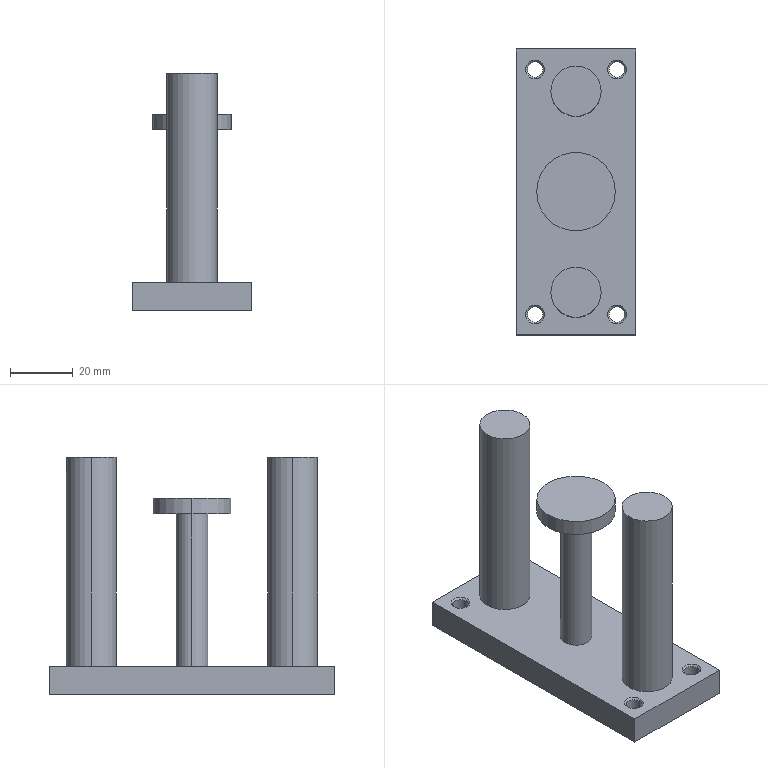Component | SolidWorks | MGPM25-30Z-M9P-1_MGPM25_30Z_0_ROD_4-1 | 1 solid | 56 faces | volume 63257 mm3 | cylinder 22 | cone 20 | plane 14 | commonest cylinder face diameters 4.917 x8 4 x6 16 x4 10 x2 25 x2